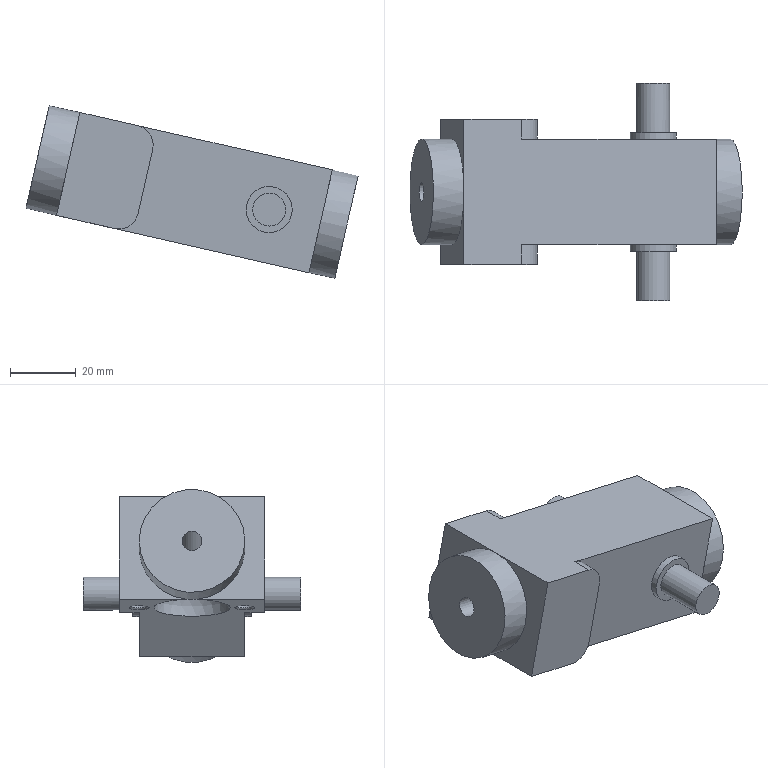Component | NX | SWING_PART | 1 solid | 40 faces | volume 73697 mm3 | plane 20 | cylinder 14 | cone 5 | sphere 1 | commonest cylinder face diameters 12 x4 32 x2 14 x2 10 x2 5 x2 24 x1 6 x1